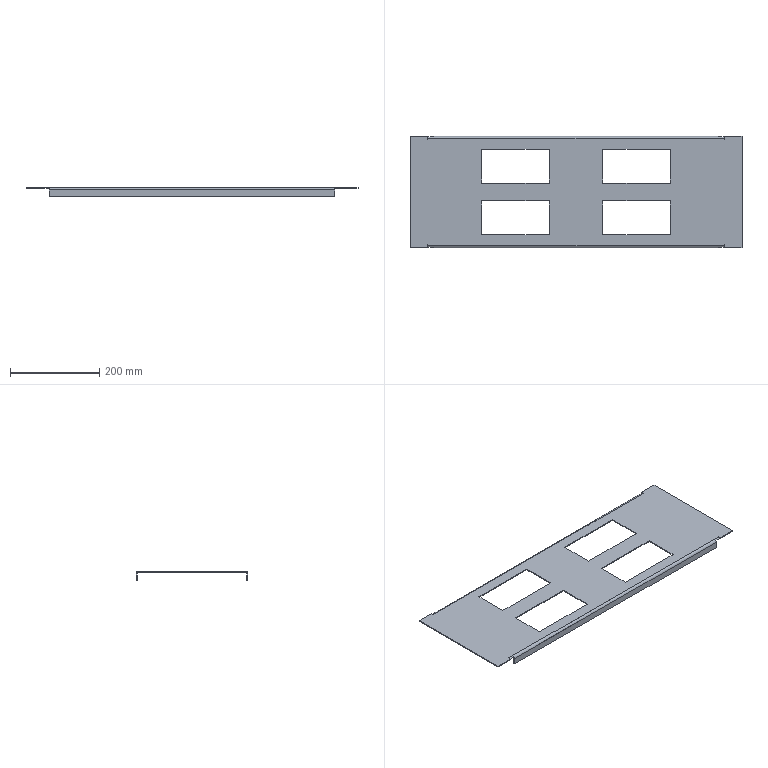Component | SolidWorks | Panel2-2 | 1 solid | 54 faces | volume 320913 mm3 | plane 50 | cylinder 4 | commonest cylinder face diameters 11 x2 7 x2 | material Plain Carbon Steel